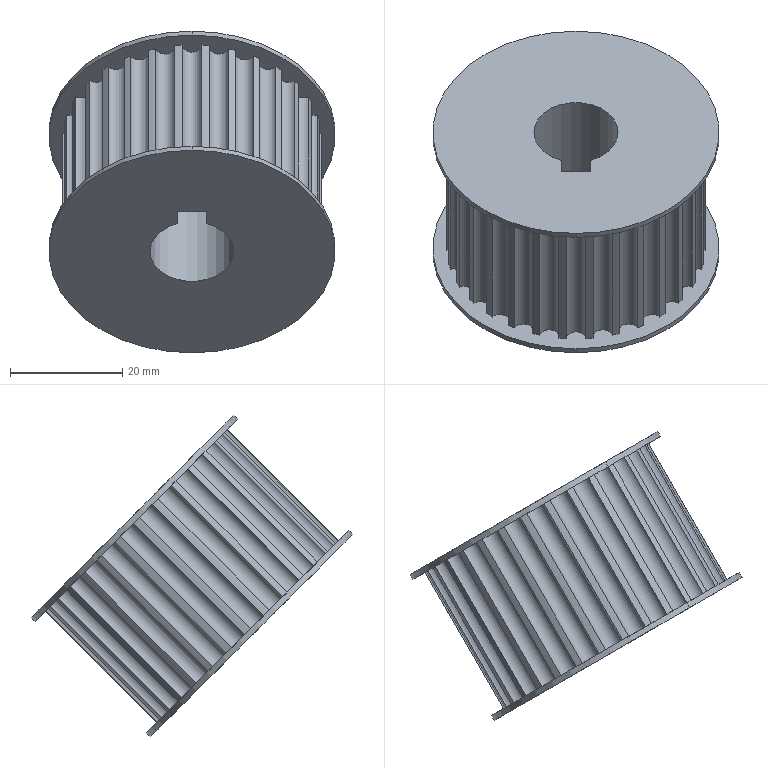Component | SolidWorks | AssemblyDriveAxis-1_InnerHole15b=5SynchronousWheel-1 | 1 solid | 87 faces | volume 40946 mm3 | cylinder 80 | plane 7 | commonest cylinder face diameters 3.5 x45 46 x30 51 x4 15 x1